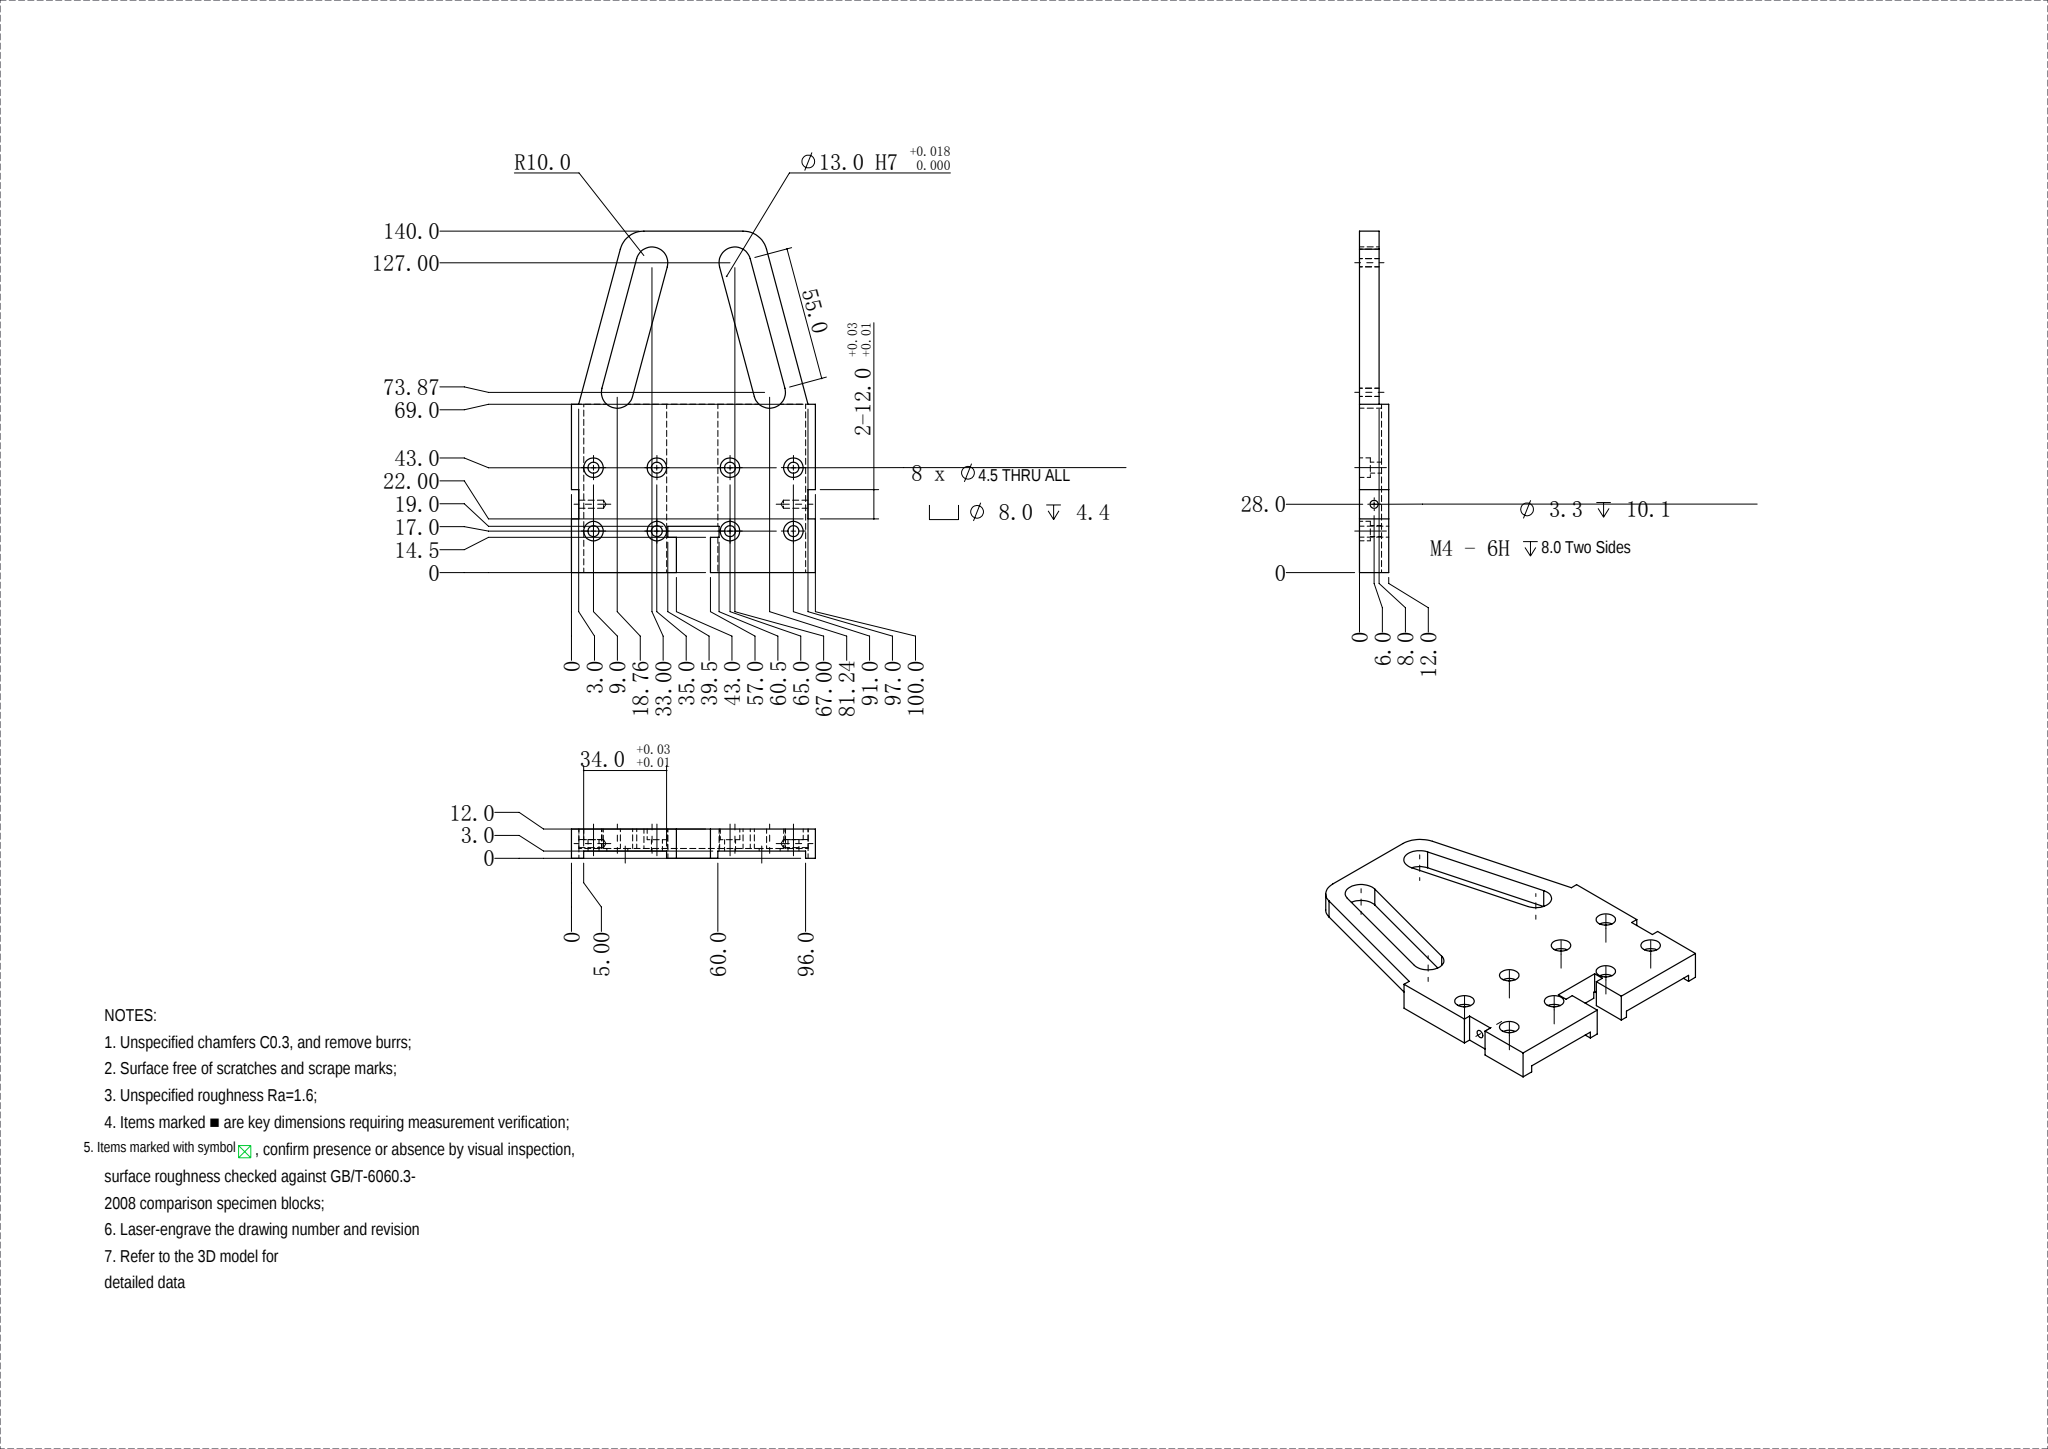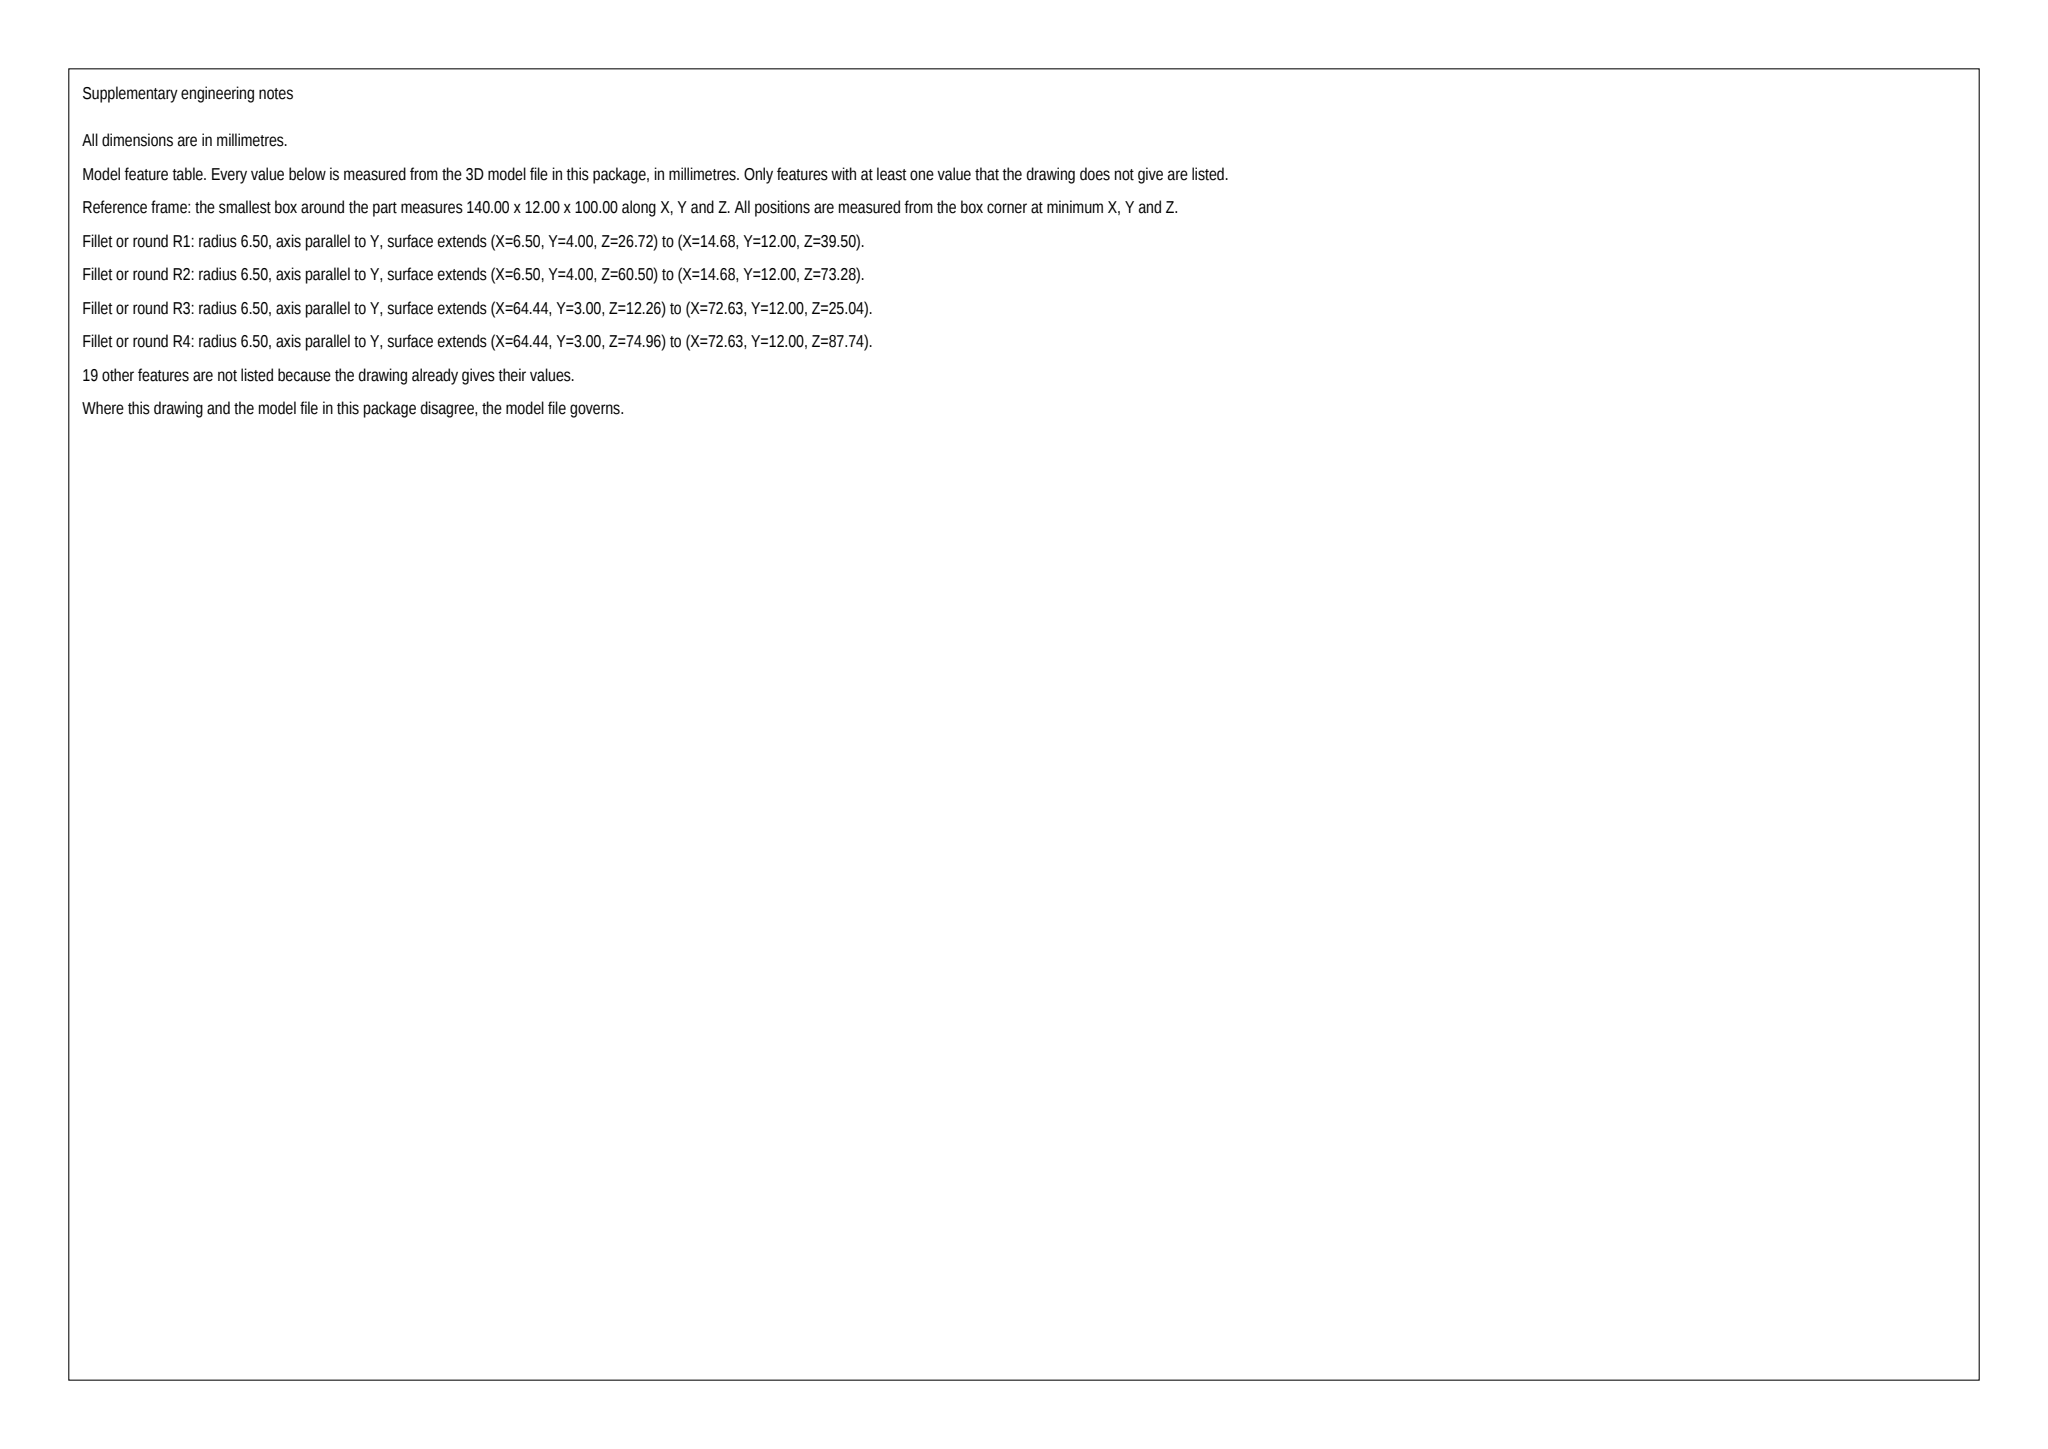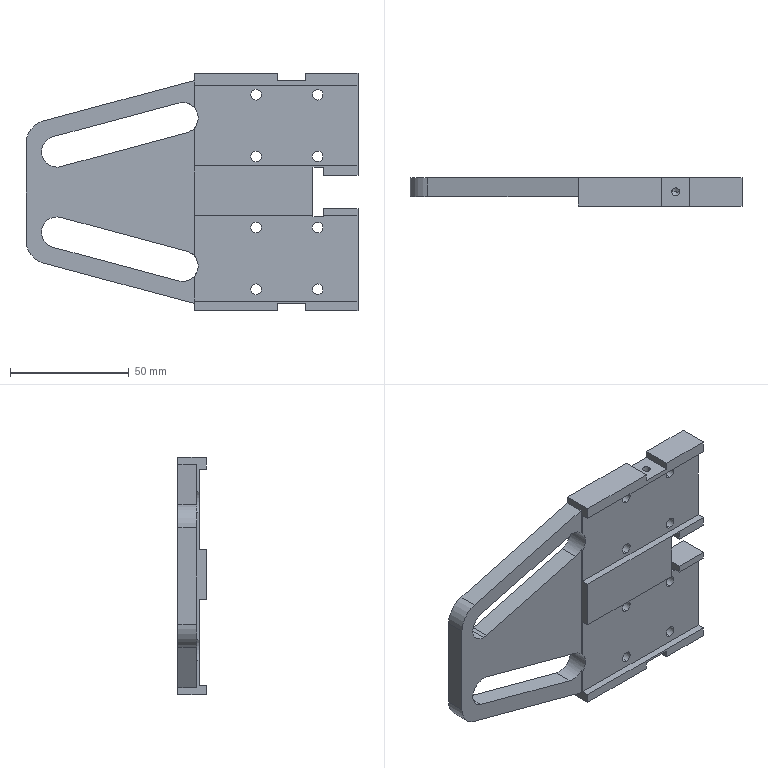Part | SolidWorks | mm | 1 solid | 98 faces | box 140 x 12 x 100 mm | volume 90200 mm3 | plane 50 | cylinder 44 | cone 4 | commonest cylinder face diameters 8 x16 4.5 x16 13 x6 3.3 x4 20 x2
Drawing notes:
STOCK 140.0 X 100.0 X 12.0 THK | from the solid: bbox_xyz [140.0, 12.0, 100.0]
2X ARM 15° FROM VERT; TIP R10.0 CTR 130.0 UP, Z29.67 & 70.33 | from the solid: Ø20 (R10) cyls axis y at x=10, z=29.67/70.33 → 140-10=130.0 up; slot axis [13,33]-[66.13,18.76] = 15°
2X ARM SLOT Ø13.0 W, DP 8.0 FROM TOP FACE, 55.0 C-C, 15° | from the solid: Ø13 cyls axis y len 8.0, ends [13,33]-[66.13,18.76] & [13,67]-[66.13,81.24]; y-plane 4.0 = 12.0-8.0 floor
FRONT STEP FACE 34.0 ABOVE BASE | from the solid: x-normal plane pair at x=106.0; 140.0-106.0=34.0 from base datum x=140
8X Ø4.5 THRU ALL; CBORE Ø8.0 DP 4.4 BOTH SIDES | from the solid: Ø4.5 len4.6 at x=97/123, z=9/35/65/91 count 2 each; Ø8.0 len4.4 count 2 each (both y faces)
4X M4-6H DP 8.0 (Ø3.3 DP 10.1), 28.0 UP, 6.0 FROM FACE, BOTH ENDS | from the solid: 4X Ø3.3 axis z len 10.1 at [x112, y6.0] → 140-112=28.0 up, 6.0 = mid of 12.0 thk; 118° drill cones
BTM STEP PKT 3.0 DP, EDGE 14.5 FROM BASE, WALLS Z40.0 & 61.0 | from the solid: y-plane 3.0 in 12.0 thk; x-plane 125.5 → 140-125.5=14.5; z-planes 40.0 (x2) & 61.0 bound pocket
build123d program:
from build123d import *

# Parameters (mm, degrees)
EXTRUDE1_DEPTH                                  = 1
SKETCH2_W                                       = 19
SKETCH2_H                                       = 1
EXTRUDE2_DEPTH                                  = 14
SKETCH3_W                                       = 69
SKETCH3_H                                       = 1
EXTRUDE3_DEPTH                                  = 14.465
SKETCH4_W                                       = 69
SKETCH4_H                                       = 1
EXTRUDE4_DEPTH                                  = 11.489
SKETCH5_W                                       = 1
SKETCH5_H                                       = 3.5
EXTRUDE5_DEPTH                                  = 4.5
SKETCH6_W                                       = 1
SKETCH6_H                                       = 3.5
EXTRUDE6_DEPTH                                  = 4.5
EXTRUDE7_START                                  = 8
EXTRUDE7_DEPTH                                  = 8
EXTRUDE8_DEPTH                                  = 3
SKETCH9_W                                       = 69
SKETCH9_H                                       = 9
EXTRUDE9_DEPTH                                  = 2.976
SKETCH10_W                                      = 69
SKETCH10_H                                      = 4
EXTRUDE10_DEPTH                                 = 3
SKETCH11_W                                      = 14.5
SKETCH11_H                                      = 3
EXTRUDE11_DEPTH                                 = 3
SKETCH12_W                                      = 69
SKETCH12_H                                      = 5
EXTRUDE12_DEPTH                                 = 3
SKETCH13_W                                      = 12
SKETCH13_H                                      = 3
EXTRUDE13_DEPTH                                 = 87.856
SKETCH14_W                                      = 12
SKETCH14_H                                      = 3
EXTRUDE14_DEPTH                                 = 87.856
M4_HEX_SOCKET_HEAD_CAP_SCREW_CBORE1_D           = 4.5
M4_HEX_SOCKET_HEAD_CAP_SCREW_CBORE1_CBORE_D     = 8
M4_HEX_SOCKET_HEAD_CAP_SCREW_CBORE1_CBORE_DEPTH = 4.4
M4_TAPPED_HOLE1_D                               = 3.3
M4_TAPPED_HOLE1_DEPTH                           = 10.1
M4_TAPPED_HOLE1_TIP                             = 0.9914
M4_TAPPED_HOLE2_D                               = 3.3
M4_TAPPED_HOLE2_DEPTH                           = 10.1
M4_TAPPED_HOLE2_TIP                             = 0.9914
FILLET1_R                                       = 10


with BuildPart() as part:
    # Sketch1 → Extrude1 (new body)
    with BuildSketch(Plane(origin=(0, 4, 0), x_dir=(1, 0, 0), z_dir=(0, 1, 0))):
        with BuildLine():
            Line((1, -35.535), (70, -35.535))
            Line((70, -35.535), (70, 35.535))
            Line((70, 35.535), (1, 35.535))
            ThreePointArc((1, 35.535), (2.626, 31.235), (1, 26.935))
            Line((1, 26.935), (1, -26.935))
            ThreePointArc((1, -26.935), (2.626, -31.235), (1, -35.535))
        make_face()
    extrude(amount=-EXTRUDE1_DEPTH)

    # Sketch2 → Extrude2 (cut)
    with BuildSketch(Plane(origin=(0, 0, -7), x_dir=(-1, 0, 0), z_dir=(0, 0, -1))):
        with Locations((-60.5, 3.5)):
            Rectangle(SKETCH2_W, SKETCH2_H)
    extrude(amount=-EXTRUDE2_DEPTH, mode=Mode.SUBTRACT)

    # Sketch3 → Extrude3 (add)
    with BuildSketch(Plane.XY.offset(35.535)):
        with Locations((35.5, 3.5)):
            Rectangle(SKETCH3_W, SKETCH3_H)
    extrude(amount=EXTRUDE3_DEPTH)

    # Sketch4 → Extrude4 (add)
    with BuildSketch(Plane(origin=(0, 0, -35.535), x_dir=(-1, 0, 0), z_dir=(0, 0, -1))):
        with Locations((-35.5, 3.5)):
            Rectangle(SKETCH4_W, SKETCH4_H)
    extrude(amount=EXTRUDE4_DEPTH)

    # Sketch5 → Extrude5 (cut)
    with BuildSketch(Plane(origin=(51, 0, 0), x_dir=(0, -1, 0), z_dir=(-1, 0, 0))):
        with Locations((-3.5, 8.75)):
            Rectangle(SKETCH5_W, SKETCH5_H)
    extrude(amount=-EXTRUDE5_DEPTH, mode=Mode.SUBTRACT)

    # Sketch6 → Extrude6 (cut)
    with BuildSketch(Plane(origin=(51, 0, 0), x_dir=(0, -1, 0), z_dir=(-1, 0, 0))):
        with Locations((-3.5, -8.75)):
            Rectangle(SKETCH6_W, SKETCH6_H)
    extrude(amount=-EXTRUDE6_DEPTH, mode=Mode.SUBTRACT)

    # Sketch7 → Extrude7 (add)
    with BuildSketch(Plane(origin=(0, 4, 0), x_dir=(-1, 0, 0), z_dir=(0, 1, 0)).offset(EXTRUDE7_START)):
        Polygon((-70, -47.024), (-70, -7), (-55.5, -7), (-55.5, -10.5), (-51, -10.5), (-51, 10.5), (-55.5, 10.5), (-55.5, 7), (-70, 7), (-70, 50), (-1, 50), (-1, 47.024), (70, 28), (70, -28), (-1, -47.024), align=None)
        with BuildLine():
            Line((58.682, 23.279), (5.556, 37.514))
            ThreePointArc((5.556, 37.514), (-2.404, 32.917), (2.192, 24.957))
            Line((2.192, 24.957), (55.318, 10.721))
            ThreePointArc((55.318, 10.721), (63.279, 15.318), (58.682, 23.279))
        make_face(mode=Mode.SUBTRACT)
        with BuildLine():
            Line((55.318, -10.721), (2.192, -24.957))
            ThreePointArc((2.192, -24.957), (-2.404, -32.917), (5.556, -37.514))
            Line((5.556, -37.514), (58.682, -23.279))
            ThreePointArc((58.682, -23.279), (63.279, -15.318), (55.318, -10.721))
        make_face(mode=Mode.SUBTRACT)
    extrude(amount=-EXTRUDE7_DEPTH)

    # Sketch8 → Extrude8 (add)
    with BuildSketch(Plane.XZ.offset(-3)):
        Polygon((55.5, 7), (55.5, 10.5), (51, 10.5), (51, -10), (1, -10), (1, 11), (70, 11), (70, 7), align=None)
    extrude(amount=EXTRUDE8_DEPTH)

    # Sketch9 → Extrude9 (add)
    with BuildSketch(Plane(origin=(0, 0, -47.024), x_dir=(-1, 0, 0), z_dir=(0, 0, -1))):
        with Locations((-35.5, 7.5)):
            Rectangle(SKETCH9_W, SKETCH9_H)
    extrude(amount=EXTRUDE9_DEPTH)

    # Sketch10 → Extrude10 (add)
    with BuildSketch(Plane.XZ.offset(-3)):
        with Locations((35.5, -48)):
            Rectangle(SKETCH10_W, SKETCH10_H)
    extrude(amount=EXTRUDE10_DEPTH)

    # Sketch11 → Extrude11 (add)
    with BuildSketch(Plane.XZ.offset(-3)):
        with Locations((62.75, -8.5)):
            Rectangle(SKETCH11_W, SKETCH11_H)
    extrude(amount=EXTRUDE11_DEPTH)

    # Sketch12 → Extrude12 (add)
    with BuildSketch(Plane.XZ.offset(-3)):
        with Locations((35.5, 47.5)):
            Rectangle(SKETCH12_W, SKETCH12_H)
    extrude(amount=EXTRUDE12_DEPTH)

    # Sketch13 → Extrude13 (cut, through all)
    with BuildSketch(Plane(origin=(0, 12, 0), x_dir=(-1, 0, 0), z_dir=(0, 1, 0))):
        with Locations((-42, -48.5)):
            Rectangle(SKETCH13_W, SKETCH13_H)
    extrude(amount=-EXTRUDE13_DEPTH, mode=Mode.SUBTRACT)

    # Sketch14 → Extrude14 (cut, through all)
    with BuildSketch(Plane.XZ):
        with Locations((42, 48.5)):
            Rectangle(SKETCH14_W, SKETCH14_H)
    extrude(amount=-EXTRUDE14_DEPTH, mode=Mode.SUBTRACT)

    # M4 Hex Socket Head Cap Screw CBORE1 (through all)
    with Locations(Plane(origin=(0, 12, 0), x_dir=(1, 0, 0), z_dir=(0, 1, 0))):
        with Locations((27, -41), (53, -41), (53, -15), (27, -15), (27, 15), (53, 15), (53, 41), (27, 41)):
            CounterBoreHole(M4_HEX_SOCKET_HEAD_CAP_SCREW_CBORE1_D / 2, M4_HEX_SOCKET_HEAD_CAP_SCREW_CBORE1_CBORE_D / 2, M4_HEX_SOCKET_HEAD_CAP_SCREW_CBORE1_CBORE_DEPTH)

    # M4 Tapped Hole1
    with Locations(Plane.XY.offset(47)):
        with Locations((42, 6)):
            Hole(M4_TAPPED_HOLE1_D / 2, depth=M4_TAPPED_HOLE1_DEPTH)
            with Locations((0, 0, -(M4_TAPPED_HOLE1_DEPTH + M4_TAPPED_HOLE1_TIP / 2))):  # 118° drill point
                Cone(0, M4_TAPPED_HOLE1_D / 2, M4_TAPPED_HOLE1_TIP, mode=Mode.SUBTRACT)

    # M4 Tapped Hole2
    with Locations(Plane(origin=(0, 0, -47), x_dir=(-1, 0, 0), z_dir=(0, 0, -1))):
        with Locations((-42, 6)):
            Hole(M4_TAPPED_HOLE2_D / 2, depth=M4_TAPPED_HOLE2_DEPTH)
            with Locations((0, 0, -(M4_TAPPED_HOLE2_DEPTH + M4_TAPPED_HOLE2_TIP / 2))):  # 118° drill point
                Cone(0, M4_TAPPED_HOLE2_D / 2, M4_TAPPED_HOLE2_TIP, mode=Mode.SUBTRACT)

    # Fillet1
    fillet1_edges = [part.edges().sort_by_distance(p)[0] for p in [
        (-70, 8, 28),
        (-70, 8, -28),
    ]]
    fillet(fillet1_edges, radius=FILLET1_R)


solid = part.part